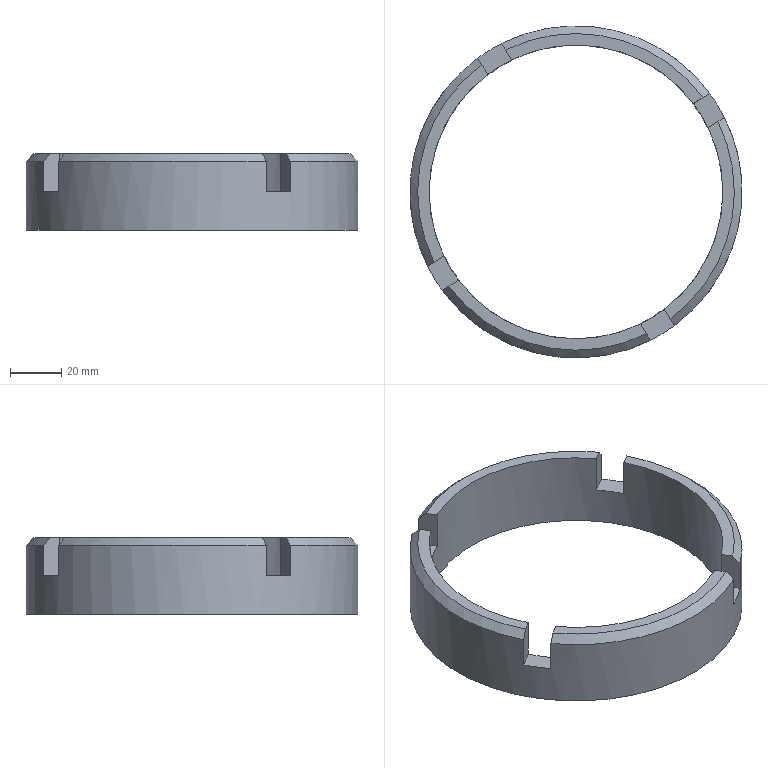Component | NX | CA6140-ZHUZHOU-MIFENG1 | 1 solid | 23 faces | volume 80023 mm3 | plane 17 | cone 4 | cylinder 2 | commonest cylinder face diameters 130 x1 115 x1